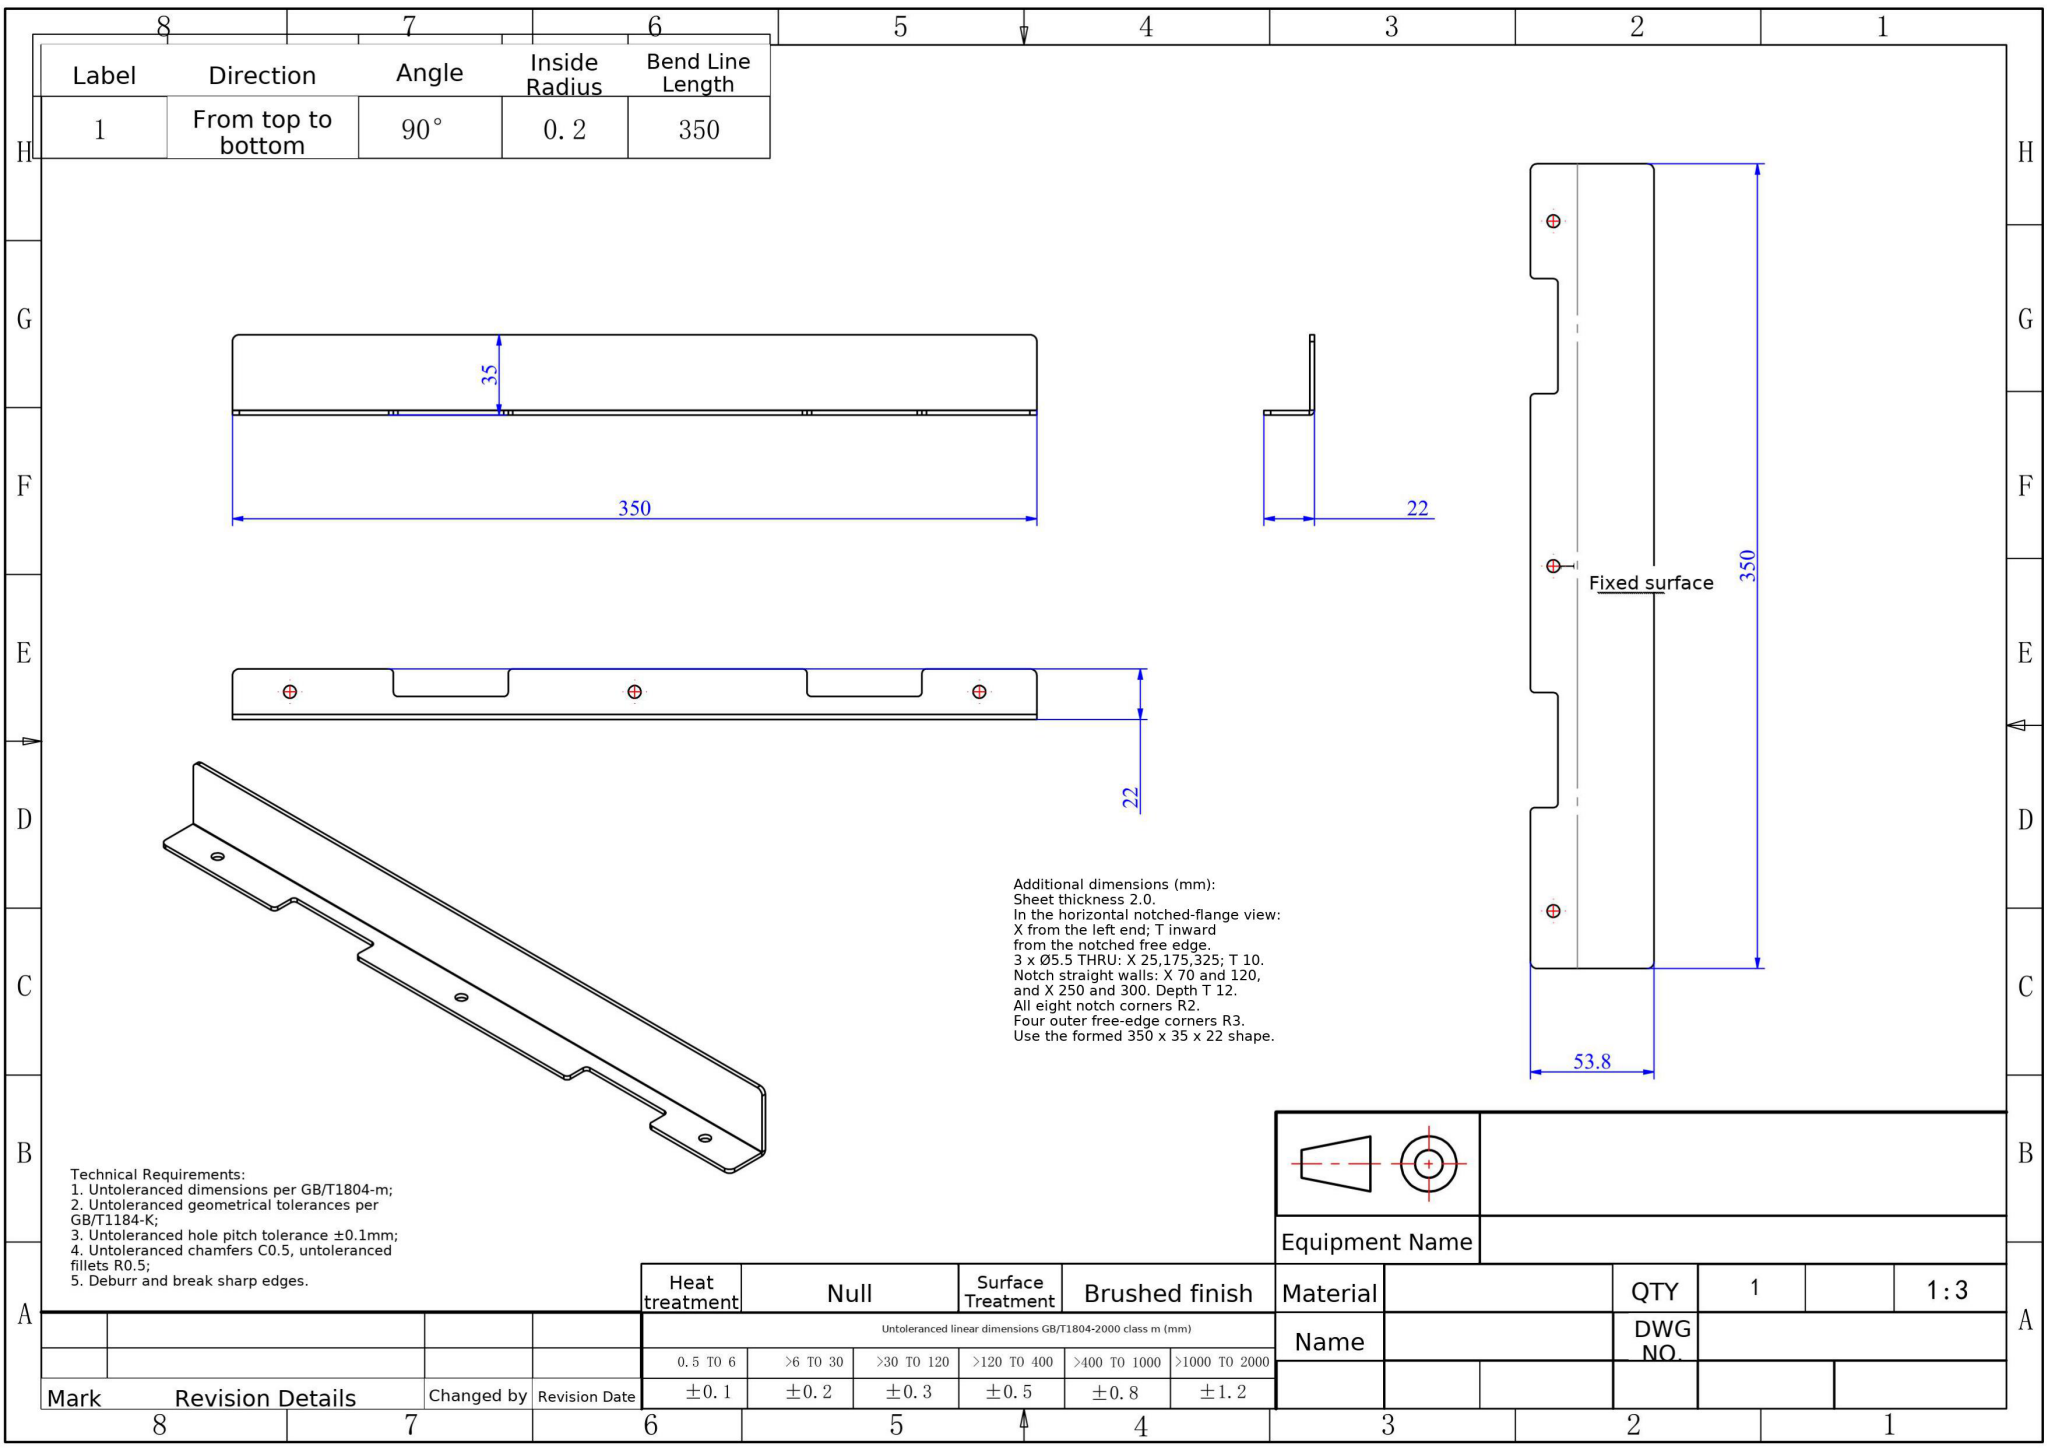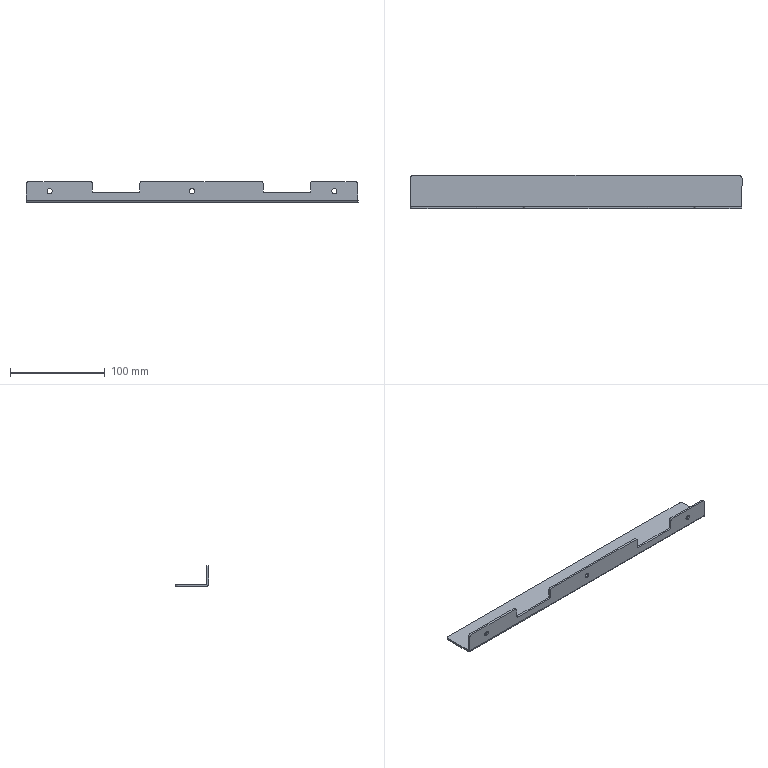Part | NX | mm | Stepped Interlocking Rail Plate | 1 solid | 40 faces | box 350 x 35 x 22 mm | volume 35581 mm3 | cylinder 20 | plane 20 | commonest cylinder face diameters 4 x8 5.5 x6 6 x4 4.4 x1 0.4 x1